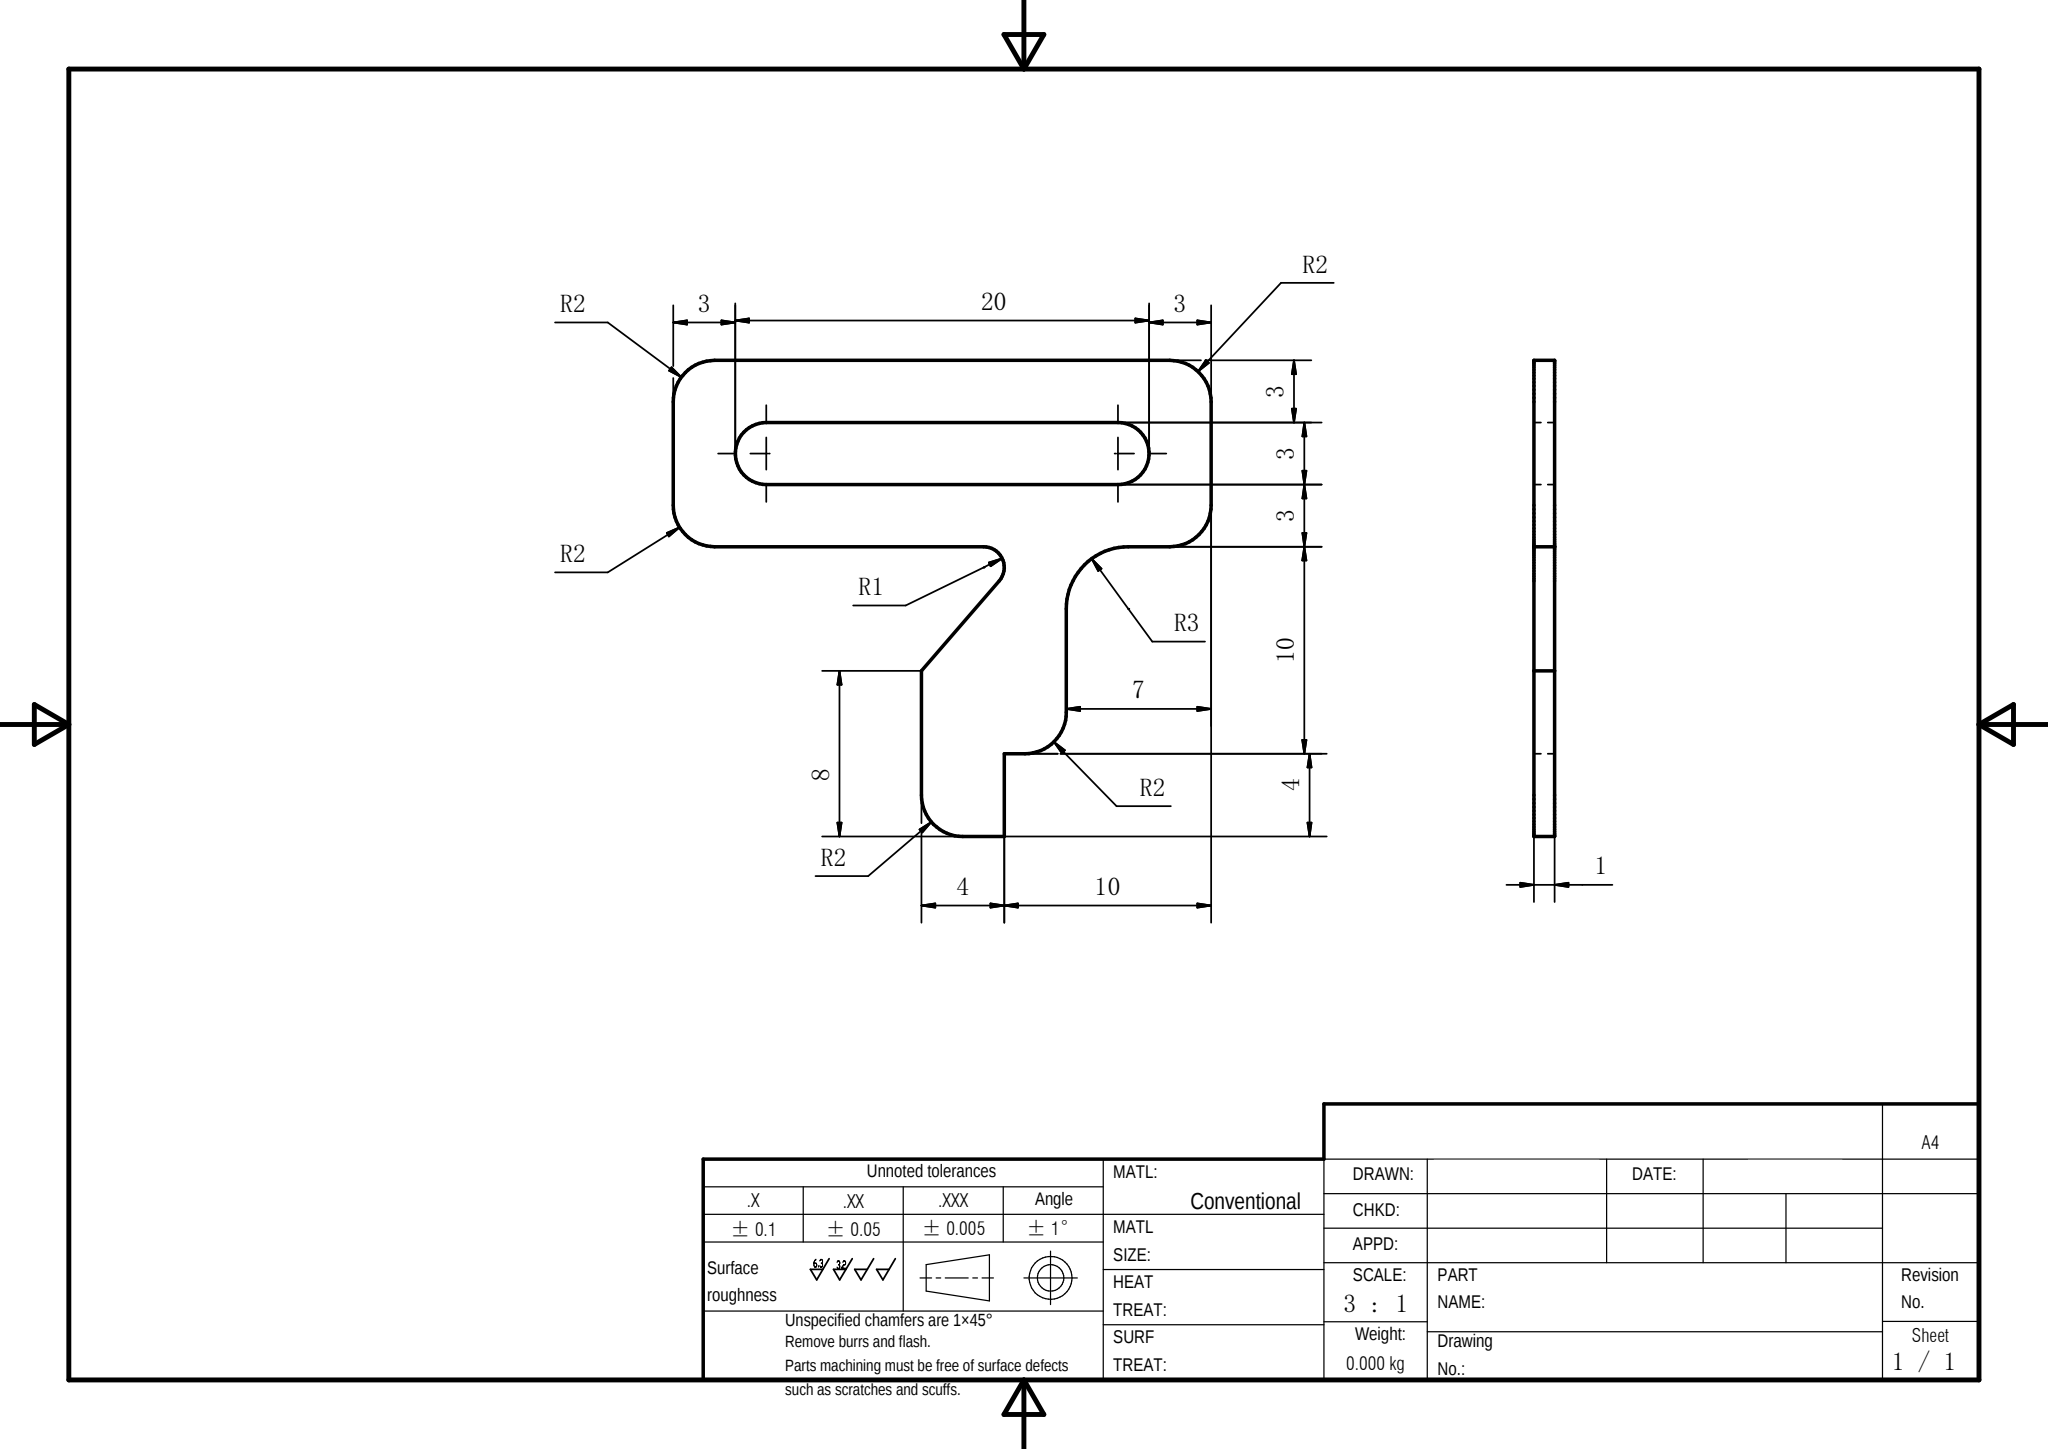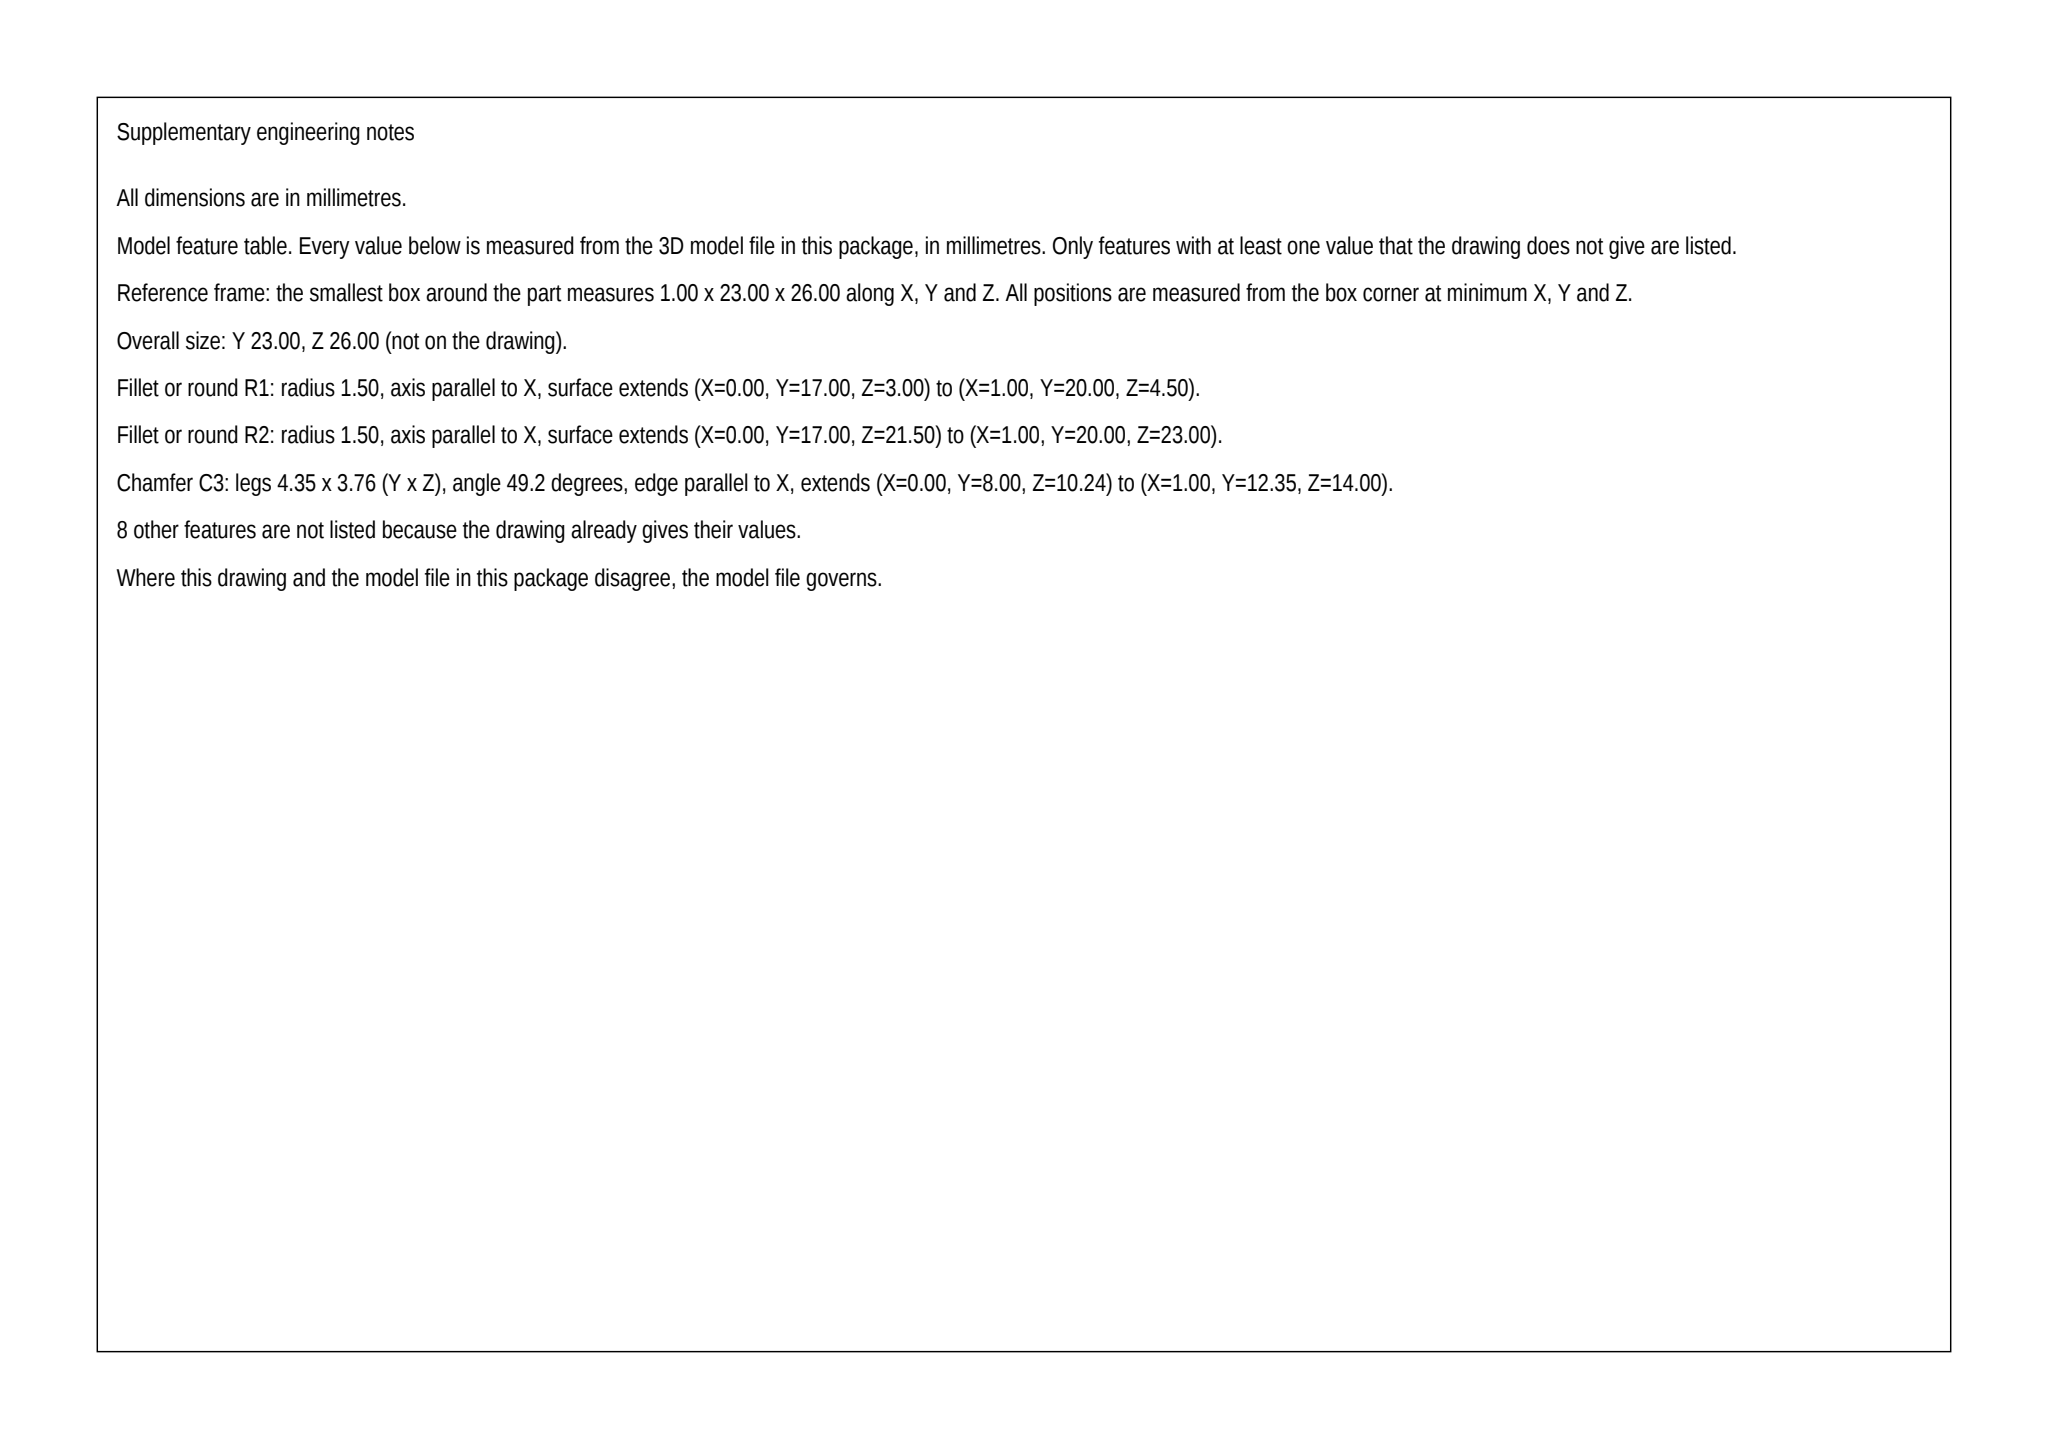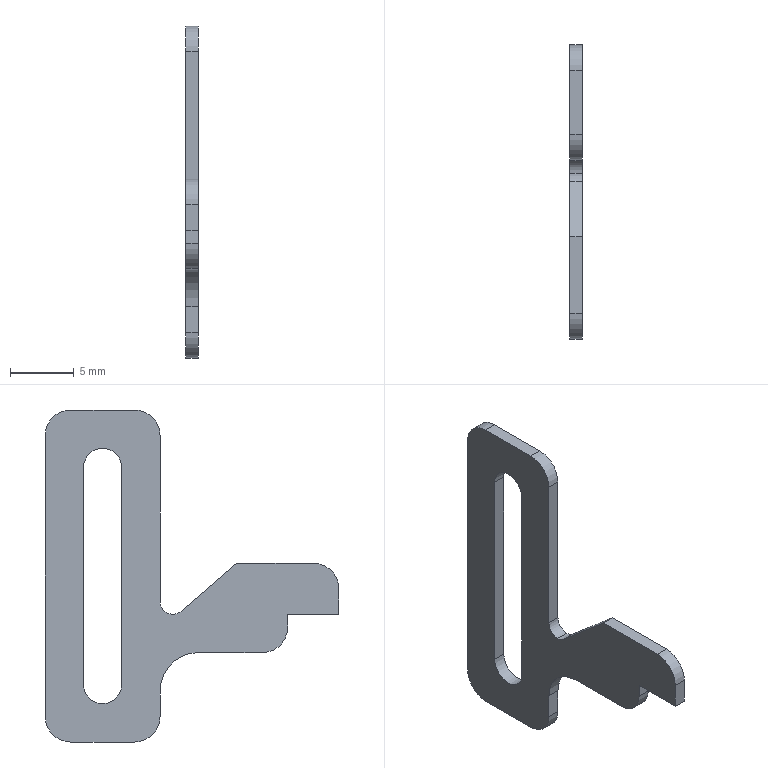Part | SolidWorks | mm | 1 solid | 27 faces | box 1 x 23 x 26 mm | volume 244 mm3 | plane 15 | cylinder 12 | commonest cylinder face diameters 4 x6 3 x3 2 x2 6 x1
STEP:
#1=CARTESIAN_POINT('',(1.,4.5,23.));
#2=VERTEX_POINT('',#1);
#3=CARTESIAN_POINT('',(1.,6.,21.5));
#4=VERTEX_POINT('',#3);
#5=CARTESIAN_POINT('',(1.,4.5,21.5));
#6=DIRECTION('',(-1.,0.,0.));
#7=DIRECTION('',(0.,0.,1.));
#8=AXIS2_PLACEMENT_3D('',#5,#6,#7);
#9=CIRCLE('',#8,1.5);
#10=EDGE_CURVE('',#2,#4,#9,.T.);
#11=ORIENTED_EDGE('',*,*,#10,.F.);
#12=CARTESIAN_POINT('',(0.,4.5,23.));
#13=VERTEX_POINT('',#12);
#14=CARTESIAN_POINT('',(1.,4.5,23.));
#15=DIRECTION('',(-1.,0.,0.));
#16=VECTOR('',#15,1000.);
#17=LINE('',#14,#16);
#18=EDGE_CURVE('',#2,#13,#17,.T.);
#19=ORIENTED_EDGE('',*,*,#18,.T.);
#20=CARTESIAN_POINT('',(0.,6.,21.5));
#21=VERTEX_POINT('',#20);
#22=CARTESIAN_POINT('',(0.,4.5,21.5));
#23=DIRECTION('',(-1.,0.,0.));
#24=DIRECTION('',(0.,0.,1.));
#25=AXIS2_PLACEMENT_3D('',#22,#23,#24);
#26=CIRCLE('',#25,1.5);
#27=EDGE_CURVE('',#13,#21,#26,.T.);
#28=ORIENTED_EDGE('',*,*,#27,.T.);
#29=CARTESIAN_POINT('',(1.,6.,21.5));
#30=DIRECTION('',(1.,0.,0.));
#31=VECTOR('',#30,1000.);
#32=LINE('',#29,#31);
#33=EDGE_CURVE('',#21,#4,#32,.T.);
#34=ORIENTED_EDGE('',*,*,#33,.T.);
#35=EDGE_LOOP('',(#11,#19,#28,#34));
#36=FACE_OUTER_BOUND('',#35,.T.);
#37=CARTESIAN_POINT('',(1.,4.5,21.5));
#38=DIRECTION('',(-1.,0.,0.));
#39=DIRECTION('',(0.,0.,1.));
#40=AXIS2_PLACEMENT_3D('',#37,#38,#39);
#41=CYLINDRICAL_SURFACE('',#40,1.5);
#42=ADVANCED_FACE('',(#36),#41,.F.);
#43=CARTESIAN_POINT('',(0.,-0.,11.));
#44=VERTEX_POINT('',#43);
#45=CARTESIAN_POINT('',(0.,-1.,10.));
#46=VERTEX_POINT('',#45);
#47=CARTESIAN_POINT('',(0.,-1.,11.));
#48=DIRECTION('',(-1.,0.,0.));
#49=DIRECTION('',(0.,0.,-1.));
#50=AXIS2_PLACEMENT_3D('',#47,#48,#49);
#51=CIRCLE('',#50,1.);
#52=EDGE_CURVE('',#44,#46,#51,.T.);
#53=ORIENTED_EDGE('',*,*,#52,.T.);
#54=CARTESIAN_POINT('',(1.,-1.,10.));
#55=VERTEX_POINT('',#54);
#56=CARTESIAN_POINT('',(0.,-1.,10.));
#57=DIRECTION('',(1.,0.,0.));
#58=VECTOR('',#57,1000.);
#59=LINE('',#56,#58);
#60=EDGE_CURVE('',#46,#55,#59,.T.);
#61=ORIENTED_EDGE('',*,*,#60,.T.);
#62=CARTESIAN_POINT('',(1.,-0.,11.));
#63=VERTEX_POINT('',#62);
#64=CARTESIAN_POINT('',(1.,-1.,11.));
#65=DIRECTION('',(-1.,0.,0.));
#66=DIRECTION('',(0.,0.,-1.));
#67=AXIS2_PLACEMENT_3D('',#64,#65,#66);
#68=CIRCLE('',#67,1.);
#69=EDGE_CURVE('',#63,#55,#68,.T.);
#70=ORIENTED_EDGE('',*,*,#69,.F.);
#71=CARTESIAN_POINT('',(0.,0.,11.));
#72=DIRECTION('',(1.,0.,0.));
#73=VECTOR('',#72,1000.);
#74=LINE('',#71,#73);
#75=EDGE_CURVE('',#44,#63,#74,.T.);
#76=ORIENTED_EDGE('',*,*,#75,.F.);
#77=EDGE_LOOP('',(#53,#61,#70,#76));
#78=FACE_OUTER_BOUND('',#77,.T.);
#79=CARTESIAN_POINT('',(0.,-1.,11.));
#80=DIRECTION('',(1.,0.,0.));
#81=DIRECTION('',(0.,0.,-1.));
#82=AXIS2_PLACEMENT_3D('',#79,#80,#81);
#83=CYLINDRICAL_SURFACE('',#82,1.);
#84=ADVANCED_FACE('',(#78),#83,.F.);
#85=CARTESIAN_POINT('',(0.,6.,4.5));
#86=VERTEX_POINT('',#85);
#87=CARTESIAN_POINT('',(0.,3.,4.5));
#88=VERTEX_POINT('',#87);
#89=CARTESIAN_POINT('',(0.,4.5,4.5));
#90=DIRECTION('',(-1.,0.,0.));
#91=DIRECTION('',(0.,0.,1.));
#92=AXIS2_PLACEMENT_3D('',#89,#90,#91);
#93=CIRCLE('',#92,1.5);
#94=EDGE_CURVE('',#86,#88,#93,.T.);
#95=ORIENTED_EDGE('',*,*,#94,.F.);
#96=CARTESIAN_POINT('',(0.,6.,13.));
#97=DIRECTION('',(0.,0.,-1.));
#98=VECTOR('',#97,1000.);
#99=LINE('',#96,#98);
#100=EDGE_CURVE('',#21,#86,#99,.T.);
#101=ORIENTED_EDGE('',*,*,#100,.F.);
#102=ORIENTED_EDGE('',*,*,#27,.F.);
#103=CARTESIAN_POINT('',(0.,3.,21.5));
#104=VERTEX_POINT('',#103);
#105=CARTESIAN_POINT('',(0.,4.5,21.5));
#106=DIRECTION('',(-1.,0.,0.));
#107=DIRECTION('',(0.,0.,1.));
#108=AXIS2_PLACEMENT_3D('',#105,#106,#107);
#109=CIRCLE('',#108,1.5);
#110=EDGE_CURVE('',#104,#13,#109,.T.);
#111=ORIENTED_EDGE('',*,*,#110,.F.);
#112=CARTESIAN_POINT('',(0.,3.,13.));
#113=DIRECTION('',(0.,0.,1.));
#114=VECTOR('',#113,1000.);
#115=LINE('',#112,#114);
#116=EDGE_CURVE('',#88,#104,#115,.T.);
#117=ORIENTED_EDGE('',*,*,#116,.F.);
#118=EDGE_LOOP('',(#95,#101,#102,#111,#117));
#119=FACE_BOUND('',#118,.T.);
#120=CARTESIAN_POINT('',(0.,7.,26.));
#121=VERTEX_POINT('',#120);
#122=CARTESIAN_POINT('',(0.,2.,26.));
#123=VERTEX_POINT('',#122);
#124=CARTESIAN_POINT('',(0.,4.5,26.));
#125=DIRECTION('',(0.,-1.,0.));
#126=VECTOR('',#125,1000.);
#127=LINE('',#124,#126);
#128=EDGE_CURVE('',#121,#123,#127,.T.);
#129=ORIENTED_EDGE('',*,*,#128,.F.);
#130=CARTESIAN_POINT('',(0.,9.,24.));
#131=VERTEX_POINT('',#130);
#132=CARTESIAN_POINT('',(0.,7.,24.));
#133=DIRECTION('',(1.,0.,0.));
#134=DIRECTION('',(0.,0.,-1.));
#135=AXIS2_PLACEMENT_3D('',#132,#133,#134);
#136=CIRCLE('',#135,2.);
#137=EDGE_CURVE('',#131,#121,#136,.T.);
#138=ORIENTED_EDGE('',*,*,#137,.F.);
#139=CARTESIAN_POINT('',(0.,9.,2.));
#140=VERTEX_POINT('',#139);
#141=CARTESIAN_POINT('',(0.,9.,13.));
#142=DIRECTION('',(0.,0.,1.));
#143=VECTOR('',#142,1000.);
#144=LINE('',#141,#143);
#145=EDGE_CURVE('',#140,#131,#144,.T.);
#146=ORIENTED_EDGE('',*,*,#145,.F.);
#147=CARTESIAN_POINT('',(0.,7.,0.));
#148=VERTEX_POINT('',#147);
#149=CARTESIAN_POINT('',(0.,7.,2.));
#150=DIRECTION('',(1.,0.,0.));
#151=DIRECTION('',(0.,0.,-1.));
#152=AXIS2_PLACEMENT_3D('',#149,#150,#151);
#153=CIRCLE('',#152,2.);
#154=EDGE_CURVE('',#148,#140,#153,.T.);
#155=ORIENTED_EDGE('',*,*,#154,.F.);
#156=CARTESIAN_POINT('',(0.,2.,0.));
#157=VERTEX_POINT('',#156);
#158=CARTESIAN_POINT('',(0.,4.5,0.));
#159=DIRECTION('',(0.,1.,0.));
#160=VECTOR('',#159,1000.);
#161=LINE('',#158,#160);
#162=EDGE_CURVE('',#157,#148,#161,.T.);
#163=ORIENTED_EDGE('',*,*,#162,.F.);
#164=CARTESIAN_POINT('',(0.,-0.,2.));
#165=VERTEX_POINT('',#164);
#166=CARTESIAN_POINT('',(0.,2.,2.));
#167=DIRECTION('',(1.,0.,0.));
#168=DIRECTION('',(0.,0.,-1.));
#169=AXIS2_PLACEMENT_3D('',#166,#167,#168);
#170=CIRCLE('',#169,2.);
#171=EDGE_CURVE('',#165,#157,#170,.T.);
#172=ORIENTED_EDGE('',*,*,#171,.F.);
#173=CARTESIAN_POINT('',(0.,-0.,4.));
#174=VERTEX_POINT('',#173);
#175=CARTESIAN_POINT('',(0.,-0.,13.));
#176=DIRECTION('',(0.,0.,-1.));
#177=VECTOR('',#176,1000.);
#178=LINE('',#175,#177);
#179=EDGE_CURVE('',#174,#165,#178,.T.);
#180=ORIENTED_EDGE('',*,*,#179,.F.);
#181=CARTESIAN_POINT('',(0.,-3.,7.));
#182=VERTEX_POINT('',#181);
#183=CARTESIAN_POINT('',(0.,-3.,4.));
#184=DIRECTION('',(-1.,0.,0.));
#185=DIRECTION('',(0.,0.,-1.));
#186=AXIS2_PLACEMENT_3D('',#183,#184,#185);
#187=CIRCLE('',#186,3.);
#188=EDGE_CURVE('',#182,#174,#187,.T.);
#189=ORIENTED_EDGE('',*,*,#188,.F.);
#190=CARTESIAN_POINT('',(0.,-8.,7.));
#191=VERTEX_POINT('',#190);
#192=CARTESIAN_POINT('',(0.,4.5,7.));
#193=DIRECTION('',(0.,1.,0.));
#194=VECTOR('',#193,1000.);
#195=LINE('',#192,#194);
#196=EDGE_CURVE('',#191,#182,#195,.T.);
#197=ORIENTED_EDGE('',*,*,#196,.F.);
#198=CARTESIAN_POINT('',(0.,-10.,9.));
#199=VERTEX_POINT('',#198);
#200=CARTESIAN_POINT('',(0.,-8.,9.));
#201=DIRECTION('',(1.,0.,0.));
#202=DIRECTION('',(0.,0.,-1.));
#203=AXIS2_PLACEMENT_3D('',#200,#201,#202);
#204=CIRCLE('',#203,2.);
#205=EDGE_CURVE('',#199,#191,#204,.T.);
#206=ORIENTED_EDGE('',*,*,#205,.F.);
#207=CARTESIAN_POINT('',(0.,-10.,10.));
#208=VERTEX_POINT('',#207);
#209=CARTESIAN_POINT('',(0.,-10.,13.));
#210=DIRECTION('',(0.,0.,-1.));
#211=VECTOR('',#210,1000.);
#212=LINE('',#209,#211);
#213=EDGE_CURVE('',#208,#199,#212,.T.);
#214=ORIENTED_EDGE('',*,*,#213,.F.);
#215=CARTESIAN_POINT('',(0.,-14.,10.));
#216=VERTEX_POINT('',#215);
#217=CARTESIAN_POINT('',(0.,4.5,10.));
#218=DIRECTION('',(0.,1.,0.));
#219=VECTOR('',#218,1000.);
#220=LINE('',#217,#219);
#221=EDGE_CURVE('',#216,#208,#220,.T.);
#222=ORIENTED_EDGE('',*,*,#221,.F.);
#223=CARTESIAN_POINT('',(0.,-14.,12.));
#224=VERTEX_POINT('',#223);
#225=CARTESIAN_POINT('',(0.,-14.,13.));
#226=DIRECTION('',(0.,0.,-1.));
#227=VECTOR('',#226,1000.);
#228=LINE('',#225,#227);
#229=EDGE_CURVE('',#224,#216,#228,.T.);
#230=ORIENTED_EDGE('',*,*,#229,.F.);
#231=CARTESIAN_POINT('',(0.,-12.,14.));
#232=VERTEX_POINT('',#231);
#233=CARTESIAN_POINT('',(0.,-12.,12.));
#234=DIRECTION('',(1.,0.,0.));
#235=DIRECTION('',(0.,0.,-1.));
#236=AXIS2_PLACEMENT_3D('',#233,#234,#235);
#237=CIRCLE('',#236,2.);
#238=EDGE_CURVE('',#232,#224,#237,.T.);
#239=ORIENTED_EDGE('',*,*,#238,.F.);
#240=CARTESIAN_POINT('',(0.,-6.,14.));
#241=VERTEX_POINT('',#240);
#242=CARTESIAN_POINT('',(0.,4.5,14.));
#243=DIRECTION('',(0.,-1.,0.));
#244=VECTOR('',#243,1000.);
#245=LINE('',#242,#244);
#246=EDGE_CURVE('',#241,#232,#245,.T.);
#247=ORIENTED_EDGE('',*,*,#246,.F.);
#248=CARTESIAN_POINT('',(0.,-1.654,10.243));
#249=VERTEX_POINT('',#248);
#250=CARTESIAN_POINT('',(0.,-1.654,10.243));
#251=DIRECTION('',(0.,-0.7566,0.6539));
#252=VECTOR('',#251,1000.);
#253=LINE('',#250,#252);
#254=EDGE_CURVE('',#249,#241,#253,.T.);
#255=ORIENTED_EDGE('',*,*,#254,.F.);
#256=CARTESIAN_POINT('',(0.,-1.,11.));
#257=DIRECTION('',(-1.,0.,0.));
#258=DIRECTION('',(0.,0.,-1.));
#259=AXIS2_PLACEMENT_3D('',#256,#257,#258);
#260=CIRCLE('',#259,1.);
#261=EDGE_CURVE('',#46,#249,#260,.T.);
#262=ORIENTED_EDGE('',*,*,#261,.F.);
#263=ORIENTED_EDGE('',*,*,#52,.F.);
#264=CARTESIAN_POINT('',(0.,-0.,24.));
#265=VERTEX_POINT('',#264);
#266=CARTESIAN_POINT('',(0.,-0.,13.));
#267=DIRECTION('',(0.,0.,-1.));
#268=VECTOR('',#267,1000.);
#269=LINE('',#266,#268);
#270=EDGE_CURVE('',#265,#44,#269,.T.);
#271=ORIENTED_EDGE('',*,*,#270,.F.);
#272=CARTESIAN_POINT('',(0.,2.,24.));
#273=DIRECTION('',(1.,0.,0.));
#274=DIRECTION('',(0.,0.,-1.));
#275=AXIS2_PLACEMENT_3D('',#272,#273,#274);
#276=CIRCLE('',#275,2.);
#277=EDGE_CURVE('',#123,#265,#276,.T.);
#278=ORIENTED_EDGE('',*,*,#277,.F.);
#279=EDGE_LOOP('',(#129,#138,#146,#155,#163,#172,#180,#189,#197,#206,#214,#222,#230,#239,#247,#255,#262,#263,#271,#278));
#280=FACE_OUTER_BOUND('',#279,.T.);
#281=CARTESIAN_POINT('',(0.,4.5,13.));
#282=DIRECTION('',(1.,0.,0.));
#283=DIRECTION('',(0.,0.,-1.));
#284=AXIS2_PLACEMENT_3D('',#281,#282,#283);
#285=PLANE('',#284);
#286=ADVANCED_FACE('',(#119,#280),#285,.F.);
#287=CARTESIAN_POINT('',(1.,3.,4.5));
#288=VERTEX_POINT('',#287);
#289=CARTESIAN_POINT('',(1.,3.,4.5));
#290=DIRECTION('',(1.,0.,0.));
#291=VECTOR('',#290,1000.);
#292=LINE('',#289,#291);
#293=EDGE_CURVE('',#88,#288,#292,.T.);
#294=ORIENTED_EDGE('',*,*,#293,.F.);
#295=ORIENTED_EDGE('',*,*,#116,.T.);
#296=CARTESIAN_POINT('',(1.,3.,21.5));
#297=VERTEX_POINT('',#296);
#298=CARTESIAN_POINT('',(1.,3.,21.5));
#299=DIRECTION('',(-1.,0.,0.));
#300=VECTOR('',#299,1000.);
#301=LINE('',#298,#300);
#302=EDGE_CURVE('',#297,#104,#301,.T.);
#303=ORIENTED_EDGE('',*,*,#302,.F.);
#304=CARTESIAN_POINT('',(1.,3.,4.5));
#305=DIRECTION('',(0.,-0.,1.));
#306=VECTOR('',#305,1000.);
#307=LINE('',#304,#306);
#308=EDGE_CURVE('',#288,#297,#307,.T.);
#309=ORIENTED_EDGE('',*,*,#308,.F.);
#310=EDGE_LOOP('',(#294,#295,#303,#309));
#311=FACE_OUTER_BOUND('',#310,.T.);
#312=CARTESIAN_POINT('',(1.,3.,4.5));
#313=DIRECTION('',(0.,-1.,-0.));
#314=DIRECTION('',(0.,0.,-1.));
#315=AXIS2_PLACEMENT_3D('',#312,#313,#314);
#316=PLANE('',#315);
#317=ADVANCED_FACE('',(#311),#316,.F.);
#318=CARTESIAN_POINT('',(1.,6.,4.5));
#319=VERTEX_POINT('',#318);
#320=CARTESIAN_POINT('',(1.,6.,4.5));
#321=DIRECTION('',(1.,0.,0.));
#322=VECTOR('',#321,1000.);
#323=LINE('',#320,#322);
#324=EDGE_CURVE('',#86,#319,#323,.T.);
#325=ORIENTED_EDGE('',*,*,#324,.F.);
#326=ORIENTED_EDGE('',*,*,#94,.T.);
#327=ORIENTED_EDGE('',*,*,#293,.T.);
#328=CARTESIAN_POINT('',(1.,4.5,4.5));
#329=DIRECTION('',(-1.,0.,0.));
#330=DIRECTION('',(0.,0.,1.));
#331=AXIS2_PLACEMENT_3D('',#328,#329,#330);
#332=CIRCLE('',#331,1.5);
#333=EDGE_CURVE('',#319,#288,#332,.T.);
#334=ORIENTED_EDGE('',*,*,#333,.F.);
#335=EDGE_LOOP('',(#325,#326,#327,#334));
#336=FACE_OUTER_BOUND('',#335,.T.);
#337=CARTESIAN_POINT('',(1.,4.5,4.5));
#338=DIRECTION('',(-1.,0.,0.));
#339=DIRECTION('',(0.,0.,1.));
#340=AXIS2_PLACEMENT_3D('',#337,#338,#339);
#341=CYLINDRICAL_SURFACE('',#340,1.5);
#342=ADVANCED_FACE('',(#336),#341,.F.);
#343=ORIENTED_EDGE('',*,*,#33,.F.);
#344=ORIENTED_EDGE('',*,*,#100,.T.);
#345=ORIENTED_EDGE('',*,*,#324,.T.);
#346=CARTESIAN_POINT('',(1.,6.,21.5));
#347=DIRECTION('',(0.,0.,-1.));
#348=VECTOR('',#347,1000.);
#349=LINE('',#346,#348);
#350=EDGE_CURVE('',#4,#319,#349,.T.);
#351=ORIENTED_EDGE('',*,*,#350,.F.);
#352=EDGE_LOOP('',(#343,#344,#345,#351));
#353=FACE_OUTER_BOUND('',#352,.T.);
#354=CARTESIAN_POINT('',(1.,6.,21.5));
#355=DIRECTION('',(0.,1.,0.));
#356=DIRECTION('',(0.,-0.,1.));
#357=AXIS2_PLACEMENT_3D('',#354,#355,#356);
#358=PLANE('',#357);
#359=ADVANCED_FACE('',(#353),#358,.F.);
#360=ORIENTED_EDGE('',*,*,#18,.F.);
#361=CARTESIAN_POINT('',(1.,4.5,21.5));
#362=DIRECTION('',(-1.,0.,0.));
#363=DIRECTION('',(0.,0.,1.));
#364=AXIS2_PLACEMENT_3D('',#361,#362,#363);
#365=CIRCLE('',#364,1.5);
#366=EDGE_CURVE('',#297,#2,#365,.T.);
#367=ORIENTED_EDGE('',*,*,#366,.F.);
#368=ORIENTED_EDGE('',*,*,#302,.T.);
#369=ORIENTED_EDGE('',*,*,#110,.T.);
#370=EDGE_LOOP('',(#360,#367,#368,#369));
#371=FACE_OUTER_BOUND('',#370,.T.);
#372=CARTESIAN_POINT('',(1.,4.5,21.5));
#373=DIRECTION('',(-1.,0.,0.));
#374=DIRECTION('',(0.,0.,1.));
#375=AXIS2_PLACEMENT_3D('',#372,#373,#374);
#376=CYLINDRICAL_SURFACE('',#375,1.5);
#377=ADVANCED_FACE('',(#371),#376,.F.);
#378=ORIENTED_EDGE('',*,*,#277,.T.);
#379=CARTESIAN_POINT('',(1.,-0.,24.));
#380=VERTEX_POINT('',#379);
#381=CARTESIAN_POINT('',(0.,-0.,24.));
#382=DIRECTION('',(1.,0.,0.));
#383=VECTOR('',#382,1000.);
#384=LINE('',#381,#383);
#385=EDGE_CURVE('',#265,#380,#384,.T.);
#386=ORIENTED_EDGE('',*,*,#385,.T.);
#387=CARTESIAN_POINT('',(1.,2.,26.));
#388=VERTEX_POINT('',#387);
#389=CARTESIAN_POINT('',(1.,2.,24.));
#390=DIRECTION('',(-1.,0.,0.));
#391=DIRECTION('',(0.,0.,-1.));
#392=AXIS2_PLACEMENT_3D('',#389,#390,#391);
#393=CIRCLE('',#392,2.);
#394=EDGE_CURVE('',#380,#388,#393,.T.);
#395=ORIENTED_EDGE('',*,*,#394,.T.);
#396=CARTESIAN_POINT('',(0.,2.,26.));
#397=DIRECTION('',(-1.,0.,0.));
#398=VECTOR('',#397,1000.);
#399=LINE('',#396,#398);
#400=EDGE_CURVE('',#388,#123,#399,.T.);
#401=ORIENTED_EDGE('',*,*,#400,.T.);
#402=EDGE_LOOP('',(#378,#386,#395,#401));
#403=FACE_OUTER_BOUND('',#402,.T.);
#404=CARTESIAN_POINT('',(0.,2.,24.));
#405=DIRECTION('',(1.,0.,0.));
#406=DIRECTION('',(0.,0.,-1.));
#407=AXIS2_PLACEMENT_3D('',#404,#405,#406);
#408=CYLINDRICAL_SURFACE('',#407,2.);
#409=ADVANCED_FACE('',(#403),#408,.T.);
#410=CARTESIAN_POINT('',(1.,7.,26.));
#411=VERTEX_POINT('',#410);
#412=CARTESIAN_POINT('',(0.,7.,26.));
#413=DIRECTION('',(-1.,0.,0.));
#414=VECTOR('',#413,1000.);
#415=LINE('',#412,#414);
#416=EDGE_CURVE('',#411,#121,#415,.T.);
#417=ORIENTED_EDGE('',*,*,#416,.T.);
#418=ORIENTED_EDGE('',*,*,#128,.T.);
#419=ORIENTED_EDGE('',*,*,#400,.F.);
#420=CARTESIAN_POINT('',(1.,9.,26.));
#421=DIRECTION('',(0.,1.,0.));
#422=VECTOR('',#421,1000.);
#423=LINE('',#420,#422);
#424=EDGE_CURVE('',#388,#411,#423,.T.);
#425=ORIENTED_EDGE('',*,*,#424,.T.);
#426=EDGE_LOOP('',(#417,#418,#419,#425));
#427=FACE_OUTER_BOUND('',#426,.T.);
#428=CARTESIAN_POINT('',(0.,9.,26.));
#429=DIRECTION('',(0.,-0.,1.));
#430=DIRECTION('',(0.,-1.,-0.));
#431=AXIS2_PLACEMENT_3D('',#428,#429,#430);
#432=PLANE('',#431);
#433=ADVANCED_FACE('',(#427),#432,.T.);
#434=ORIENTED_EDGE('',*,*,#137,.T.);
#435=ORIENTED_EDGE('',*,*,#416,.F.);
#436=CARTESIAN_POINT('',(1.,9.,24.));
#437=VERTEX_POINT('',#436);
#438=CARTESIAN_POINT('',(1.,7.,24.));
#439=DIRECTION('',(-1.,0.,0.));
#440=DIRECTION('',(0.,0.,-1.));
#441=AXIS2_PLACEMENT_3D('',#438,#439,#440);
#442=CIRCLE('',#441,2.);
#443=EDGE_CURVE('',#411,#437,#442,.T.);
#444=ORIENTED_EDGE('',*,*,#443,.T.);
#445=CARTESIAN_POINT('',(0.,9.,24.));
#446=DIRECTION('',(-1.,0.,0.));
#447=VECTOR('',#446,1000.);
#448=LINE('',#445,#447);
#449=EDGE_CURVE('',#437,#131,#448,.T.);
#450=ORIENTED_EDGE('',*,*,#449,.T.);
#451=EDGE_LOOP('',(#434,#435,#444,#450));
#452=FACE_OUTER_BOUND('',#451,.T.);
#453=CARTESIAN_POINT('',(0.,7.,24.));
#454=DIRECTION('',(1.,0.,0.));
#455=DIRECTION('',(0.,0.,-1.));
#456=AXIS2_PLACEMENT_3D('',#453,#454,#455);
#457=CYLINDRICAL_SURFACE('',#456,2.);
#458=ADVANCED_FACE('',(#452),#457,.T.);
#459=CARTESIAN_POINT('',(1.,9.,2.));
#460=VERTEX_POINT('',#459);
#461=CARTESIAN_POINT('',(0.,9.,2.));
#462=DIRECTION('',(-1.,0.,0.));
#463=VECTOR('',#462,1000.);
#464=LINE('',#461,#463);
#465=EDGE_CURVE('',#460,#140,#464,.T.);
#466=ORIENTED_EDGE('',*,*,#465,.T.);
#467=ORIENTED_EDGE('',*,*,#145,.T.);
#468=ORIENTED_EDGE('',*,*,#449,.F.);
#469=CARTESIAN_POINT('',(1.,9.,0.));
#470=DIRECTION('',(0.,0.,-1.));
#471=VECTOR('',#470,1000.);
#472=LINE('',#469,#471);
#473=EDGE_CURVE('',#437,#460,#472,.T.);
#474=ORIENTED_EDGE('',*,*,#473,.T.);
#475=EDGE_LOOP('',(#466,#467,#468,#474));
#476=FACE_OUTER_BOUND('',#475,.T.);
#477=CARTESIAN_POINT('',(0.,9.,0.));
#478=DIRECTION('',(0.,1.,0.));
#479=DIRECTION('',(0.,-0.,1.));
#480=AXIS2_PLACEMENT_3D('',#477,#478,#479);
#481=PLANE('',#480);
#482=ADVANCED_FACE('',(#476),#481,.T.);
#483=ORIENTED_EDGE('',*,*,#154,.T.);
#484=ORIENTED_EDGE('',*,*,#465,.F.);
#485=CARTESIAN_POINT('',(1.,7.,0.));
#486=VERTEX_POINT('',#485);
#487=CARTESIAN_POINT('',(1.,7.,2.));
#488=DIRECTION('',(-1.,0.,0.));
#489=DIRECTION('',(0.,0.,-1.));
#490=AXIS2_PLACEMENT_3D('',#487,#488,#489);
#491=CIRCLE('',#490,2.);
#492=EDGE_CURVE('',#460,#486,#491,.T.);
#493=ORIENTED_EDGE('',*,*,#492,.T.);
#494=CARTESIAN_POINT('',(0.,7.,0.));
#495=DIRECTION('',(-1.,0.,0.));
#496=VECTOR('',#495,1000.);
#497=LINE('',#494,#496);
#498=EDGE_CURVE('',#486,#148,#497,.T.);
#499=ORIENTED_EDGE('',*,*,#498,.T.);
#500=EDGE_LOOP('',(#483,#484,#493,#499));
#501=FACE_OUTER_BOUND('',#500,.T.);
#502=CARTESIAN_POINT('',(0.,7.,2.));
#503=DIRECTION('',(1.,0.,0.));
#504=DIRECTION('',(0.,0.,-1.));
#505=AXIS2_PLACEMENT_3D('',#502,#503,#504);
#506=CYLINDRICAL_SURFACE('',#505,2.);
#507=ADVANCED_FACE('',(#501),#506,.T.);
#508=CARTESIAN_POINT('',(1.,2.,0.));
#509=VERTEX_POINT('',#508);
#510=CARTESIAN_POINT('',(0.,2.,0.));
#511=DIRECTION('',(-1.,0.,0.));
#512=VECTOR('',#511,1000.);
#513=LINE('',#510,#512);
#514=EDGE_CURVE('',#509,#157,#513,.T.);
#515=ORIENTED_EDGE('',*,*,#514,.T.);
#516=ORIENTED_EDGE('',*,*,#162,.T.);
#517=ORIENTED_EDGE('',*,*,#498,.F.);
#518=CARTESIAN_POINT('',(1.,0.,0.));
#519=DIRECTION('',(0.,-1.,0.));
#520=VECTOR('',#519,1000.);
#521=LINE('',#518,#520);
#522=EDGE_CURVE('',#486,#509,#521,.T.);
#523=ORIENTED_EDGE('',*,*,#522,.T.);
#524=EDGE_LOOP('',(#515,#516,#517,#523));
#525=FACE_OUTER_BOUND('',#524,.T.);
#526=CARTESIAN_POINT('',(0.,0.,0.));
#527=DIRECTION('',(0.,0.,-1.));
#528=DIRECTION('',(-1.,0.,0.));
#529=AXIS2_PLACEMENT_3D('',#526,#527,#528);
#530=PLANE('',#529);
#531=ADVANCED_FACE('',(#525),#530,.T.);
#532=ORIENTED_EDGE('',*,*,#171,.T.);
#533=ORIENTED_EDGE('',*,*,#514,.F.);
#534=CARTESIAN_POINT('',(1.,-0.,2.));
#535=VERTEX_POINT('',#534);
#536=CARTESIAN_POINT('',(1.,2.,2.));
#537=DIRECTION('',(-1.,0.,0.));
#538=DIRECTION('',(0.,0.,-1.));
#539=AXIS2_PLACEMENT_3D('',#536,#537,#538);
#540=CIRCLE('',#539,2.);
#541=EDGE_CURVE('',#509,#535,#540,.T.);
#542=ORIENTED_EDGE('',*,*,#541,.T.);
#543=CARTESIAN_POINT('',(0.,0.,2.));
#544=DIRECTION('',(-1.,0.,0.));
#545=VECTOR('',#544,1000.);
#546=LINE('',#543,#545);
#547=EDGE_CURVE('',#535,#165,#546,.T.);
#548=ORIENTED_EDGE('',*,*,#547,.T.);
#549=EDGE_LOOP('',(#532,#533,#542,#548));
#550=FACE_OUTER_BOUND('',#549,.T.);
#551=CARTESIAN_POINT('',(0.,2.,2.));
#552=DIRECTION('',(1.,0.,0.));
#553=DIRECTION('',(0.,0.,-1.));
#554=AXIS2_PLACEMENT_3D('',#551,#552,#553);
#555=CYLINDRICAL_SURFACE('',#554,2.);
#556=ADVANCED_FACE('',(#550),#555,.T.);
#557=ORIENTED_EDGE('',*,*,#547,.F.);
#558=CARTESIAN_POINT('',(1.,-0.,4.));
#559=VERTEX_POINT('',#558);
#560=CARTESIAN_POINT('',(1.,-0.,7.));
#561=DIRECTION('',(0.,-0.,1.));
#562=VECTOR('',#561,1000.);
#563=LINE('',#560,#562);
#564=EDGE_CURVE('',#535,#559,#563,.T.);
#565=ORIENTED_EDGE('',*,*,#564,.T.);
#566=CARTESIAN_POINT('',(0.,-0.,4.));
#567=DIRECTION('',(-1.,0.,0.));
#568=VECTOR('',#567,1000.);
#569=LINE('',#566,#568);
#570=EDGE_CURVE('',#559,#174,#569,.T.);
#571=ORIENTED_EDGE('',*,*,#570,.T.);
#572=ORIENTED_EDGE('',*,*,#179,.T.);
#573=EDGE_LOOP('',(#557,#565,#571,#572));
#574=FACE_OUTER_BOUND('',#573,.T.);
#575=CARTESIAN_POINT('',(0.,-0.,7.));
#576=DIRECTION('',(0.,-1.,-0.));
#577=DIRECTION('',(0.,0.,-1.));
#578=AXIS2_PLACEMENT_3D('',#575,#576,#577);
#579=PLANE('',#578);
#580=ADVANCED_FACE('',(#574),#579,.T.);
#581=ORIENTED_EDGE('',*,*,#570,.F.);
#582=CARTESIAN_POINT('',(1.,-3.,7.));
#583=VERTEX_POINT('',#582);
#584=CARTESIAN_POINT('',(1.,-3.,4.));
#585=DIRECTION('',(-1.,0.,0.));
#586=DIRECTION('',(0.,0.,-1.));
#587=AXIS2_PLACEMENT_3D('',#584,#585,#586);
#588=CIRCLE('',#587,3.);
#589=EDGE_CURVE('',#583,#559,#588,.T.);
#590=ORIENTED_EDGE('',*,*,#589,.F.);
#591=CARTESIAN_POINT('',(0.,-3.,7.));
#592=DIRECTION('',(1.,0.,0.));
#593=VECTOR('',#592,1000.);
#594=LINE('',#591,#593);
#595=EDGE_CURVE('',#182,#583,#594,.T.);
#596=ORIENTED_EDGE('',*,*,#595,.F.);
#597=ORIENTED_EDGE('',*,*,#188,.T.);
#598=EDGE_LOOP('',(#581,#590,#596,#597));
#599=FACE_OUTER_BOUND('',#598,.T.);
#600=CARTESIAN_POINT('',(0.,-3.,4.));
#601=DIRECTION('',(1.,0.,0.));
#602=DIRECTION('',(0.,0.,-1.));
#603=AXIS2_PLACEMENT_3D('',#600,#601,#602);
#604=CYLINDRICAL_SURFACE('',#603,3.);
#605=ADVANCED_FACE('',(#599),#604,.F.);
#606=CARTESIAN_POINT('',(1.,-8.,7.));
#607=VERTEX_POINT('',#606);
#608=CARTESIAN_POINT('',(0.,-8.,7.));
#609=DIRECTION('',(-1.,0.,0.));
#610=VECTOR('',#609,1000.);
#611=LINE('',#608,#610);
#612=EDGE_CURVE('',#607,#191,#611,.T.);
#613=ORIENTED_EDGE('',*,*,#612,.T.);
#614=ORIENTED_EDGE('',*,*,#196,.T.);
#615=ORIENTED_EDGE('',*,*,#595,.T.);
#616=CARTESIAN_POINT('',(1.,-10.,7.));
#617=DIRECTION('',(0.,-1.,-0.));
#618=VECTOR('',#617,1000.);
#619=LINE('',#616,#618);
#620=EDGE_CURVE('',#583,#607,#619,.T.);
#621=ORIENTED_EDGE('',*,*,#620,.T.);
#622=EDGE_LOOP('',(#613,#614,#615,#621));
#623=FACE_OUTER_BOUND('',#622,.T.);
#624=CARTESIAN_POINT('',(0.,-10.,7.));
#625=DIRECTION('',(0.,0.,-1.));
#626=DIRECTION('',(0.,1.,0.));
#627=AXIS2_PLACEMENT_3D('',#624,#625,#626);
#628=PLANE('',#627);
#629=ADVANCED_FACE('',(#623),#628,.T.);
#630=ORIENTED_EDGE('',*,*,#205,.T.);
#631=ORIENTED_EDGE('',*,*,#612,.F.);
#632=CARTESIAN_POINT('',(1.,-10.,9.));
#633=VERTEX_POINT('',#632);
#634=CARTESIAN_POINT('',(1.,-8.,9.));
#635=DIRECTION('',(-1.,0.,0.));
#636=DIRECTION('',(0.,0.,-1.));
#637=AXIS2_PLACEMENT_3D('',#634,#635,#636);
#638=CIRCLE('',#637,2.);
#639=EDGE_CURVE('',#607,#633,#638,.T.);
#640=ORIENTED_EDGE('',*,*,#639,.T.);
#641=CARTESIAN_POINT('',(0.,-10.,9.));
#642=DIRECTION('',(-1.,0.,0.));
#643=VECTOR('',#642,1000.);
#644=LINE('',#641,#643);
#645=EDGE_CURVE('',#633,#199,#644,.T.);
#646=ORIENTED_EDGE('',*,*,#645,.T.);
#647=EDGE_LOOP('',(#630,#631,#640,#646));
#648=FACE_OUTER_BOUND('',#647,.T.);
#649=CARTESIAN_POINT('',(0.,-8.,9.));
#650=DIRECTION('',(1.,0.,0.));
#651=DIRECTION('',(0.,0.,-1.));
#652=AXIS2_PLACEMENT_3D('',#649,#650,#651);
#653=CYLINDRICAL_SURFACE('',#652,2.);
#654=ADVANCED_FACE('',(#648),#653,.T.);
#655=CARTESIAN_POINT('',(1.,-10.,10.));
#656=VERTEX_POINT('',#655);
#657=CARTESIAN_POINT('',(0.,-10.,10.));
#658=DIRECTION('',(-1.,0.,0.));
#659=VECTOR('',#658,1000.);
#660=LINE('',#657,#659);
#661=EDGE_CURVE('',#656,#208,#660,.T.);
#662=ORIENTED_EDGE('',*,*,#661,.T.);
#663=ORIENTED_EDGE('',*,*,#213,.T.);
#664=ORIENTED_EDGE('',*,*,#645,.F.);
#665=CARTESIAN_POINT('',(1.,-10.,10.));
#666=DIRECTION('',(0.,0.,1.));
#667=VECTOR('',#666,1000.);
#668=LINE('',#665,#667);
#669=EDGE_CURVE('',#633,#656,#668,.T.);
#670=ORIENTED_EDGE('',*,*,#669,.T.);
#671=EDGE_LOOP('',(#662,#663,#664,#670));
#672=FACE_OUTER_BOUND('',#671,.T.);
#673=CARTESIAN_POINT('',(0.,-10.,10.));
#674=DIRECTION('',(0.,-1.,0.));
#675=DIRECTION('',(0.,0.,-1.));
#676=AXIS2_PLACEMENT_3D('',#673,#674,#675);
#677=PLANE('',#676);
#678=ADVANCED_FACE('',(#672),#677,.T.);
#679=CARTESIAN_POINT('',(1.,-14.,10.));
#680=VERTEX_POINT('',#679);
#681=CARTESIAN_POINT('',(1.,-14.,10.));
#682=DIRECTION('',(0.,-1.,0.));
#683=VECTOR('',#682,1000.);
#684=LINE('',#681,#683);
#685=EDGE_CURVE('',#656,#680,#684,.T.);
#686=ORIENTED_EDGE('',*,*,#685,.T.);
#687=CARTESIAN_POINT('',(0.,-14.,10.));
#688=DIRECTION('',(-1.,0.,0.));
#689=VECTOR('',#688,1000.);
#690=LINE('',#687,#689);
#691=EDGE_CURVE('',#680,#216,#690,.T.);
#692=ORIENTED_EDGE('',*,*,#691,.T.);
#693=ORIENTED_EDGE('',*,*,#221,.T.);
#694=ORIENTED_EDGE('',*,*,#661,.F.);
#695=EDGE_LOOP('',(#686,#692,#693,#694));
#696=FACE_OUTER_BOUND('',#695,.T.);
#697=CARTESIAN_POINT('',(0.,-14.,10.));
#698=DIRECTION('',(0.,0.,-1.));
#699=DIRECTION('',(-1.,0.,0.));
#700=AXIS2_PLACEMENT_3D('',#697,#698,#699);
#701=PLANE('',#700);
#702=ADVANCED_FACE('',(#696),#701,.T.);
#703=ORIENTED_EDGE('',*,*,#691,.F.);
#704=CARTESIAN_POINT('',(1.,-14.,12.));
#705=VERTEX_POINT('',#704);
#706=CARTESIAN_POINT('',(1.,-14.,14.));
#707=DIRECTION('',(0.,-0.,1.));
#708=VECTOR('',#707,1000.);
#709=LINE('',#706,#708);
#710=EDGE_CURVE('',#680,#705,#709,.T.);
#711=ORIENTED_EDGE('',*,*,#710,.T.);
#712=CARTESIAN_POINT('',(0.,-14.,12.));
#713=DIRECTION('',(-1.,0.,0.));
#714=VECTOR('',#713,1000.);
#715=LINE('',#712,#714);
#716=EDGE_CURVE('',#705,#224,#715,.T.);
#717=ORIENTED_EDGE('',*,*,#716,.T.);
#718=ORIENTED_EDGE('',*,*,#229,.T.);
#719=EDGE_LOOP('',(#703,#711,#717,#718));
#720=FACE_OUTER_BOUND('',#719,.T.);
#721=CARTESIAN_POINT('',(0.,-14.,14.));
#722=DIRECTION('',(0.,-1.,-0.));
#723=DIRECTION('',(0.,0.,-1.));
#724=AXIS2_PLACEMENT_3D('',#721,#722,#723);
#725=PLANE('',#724);
#726=ADVANCED_FACE('',(#720),#725,.T.);
#727=ORIENTED_EDGE('',*,*,#238,.T.);
#728=ORIENTED_EDGE('',*,*,#716,.F.);
#729=CARTESIAN_POINT('',(1.,-12.,14.));
#730=VERTEX_POINT('',#729);
#731=CARTESIAN_POINT('',(1.,-12.,12.));
#732=DIRECTION('',(-1.,0.,0.));
#733=DIRECTION('',(0.,0.,-1.));
#734=AXIS2_PLACEMENT_3D('',#731,#732,#733);
#735=CIRCLE('',#734,2.);
#736=EDGE_CURVE('',#705,#730,#735,.T.);
#737=ORIENTED_EDGE('',*,*,#736,.T.);
#738=CARTESIAN_POINT('',(0.,-12.,14.));
#739=DIRECTION('',(-1.,0.,0.));
#740=VECTOR('',#739,1000.);
#741=LINE('',#738,#740);
#742=EDGE_CURVE('',#730,#232,#741,.T.);
#743=ORIENTED_EDGE('',*,*,#742,.T.);
#744=EDGE_LOOP('',(#727,#728,#737,#743));
#745=FACE_OUTER_BOUND('',#744,.T.);
#746=CARTESIAN_POINT('',(0.,-12.,12.));
#747=DIRECTION('',(1.,0.,0.));
#748=DIRECTION('',(0.,0.,-1.));
#749=AXIS2_PLACEMENT_3D('',#746,#747,#748);
#750=CYLINDRICAL_SURFACE('',#749,2.);
#751=ADVANCED_FACE('',(#745),#750,.T.);
#752=CARTESIAN_POINT('',(1.,-6.,14.));
#753=VERTEX_POINT('',#752);
#754=CARTESIAN_POINT('',(0.,-6.,14.));
#755=DIRECTION('',(-1.,0.,0.));
#756=VECTOR('',#755,1000.);
#757=LINE('',#754,#756);
#758=EDGE_CURVE('',#753,#241,#757,.T.);
#759=ORIENTED_EDGE('',*,*,#758,.T.);
#760=ORIENTED_EDGE('',*,*,#246,.T.);
#761=ORIENTED_EDGE('',*,*,#742,.F.);
#762=CARTESIAN_POINT('',(1.,-6.,14.));
#763=DIRECTION('',(0.,1.,0.));
#764=VECTOR('',#763,1000.);
#765=LINE('',#762,#764);
#766=EDGE_CURVE('',#730,#753,#765,.T.);
#767=ORIENTED_EDGE('',*,*,#766,.T.);
#768=EDGE_LOOP('',(#759,#760,#761,#767));
#769=FACE_OUTER_BOUND('',#768,.T.);
#770=CARTESIAN_POINT('',(0.,-6.,14.));
#771=DIRECTION('',(0.,-0.,1.));
#772=DIRECTION('',(0.,-1.,-0.));
#773=AXIS2_PLACEMENT_3D('',#770,#771,#772);
#774=PLANE('',#773);
#775=ADVANCED_FACE('',(#769),#774,.T.);
#776=CARTESIAN_POINT('',(1.,-1.654,10.243));
#777=VERTEX_POINT('',#776);
#778=CARTESIAN_POINT('',(1.,-1.654,10.243));
#779=DIRECTION('',(0.,0.7566,-0.6539));
#780=VECTOR('',#779,1000.);
#781=LINE('',#778,#780);
#782=EDGE_CURVE('',#753,#777,#781,.T.);
#783=ORIENTED_EDGE('',*,*,#782,.T.);
#784=CARTESIAN_POINT('',(0.,-1.654,10.243));
#785=DIRECTION('',(-1.,0.,0.));
#786=VECTOR('',#785,1000.);
#787=LINE('',#784,#786);
#788=EDGE_CURVE('',#777,#249,#787,.T.);
#789=ORIENTED_EDGE('',*,*,#788,.T.);
#790=ORIENTED_EDGE('',*,*,#254,.T.);
#791=ORIENTED_EDGE('',*,*,#758,.F.);
#792=EDGE_LOOP('',(#783,#789,#790,#791));
#793=FACE_OUTER_BOUND('',#792,.T.);
#794=CARTESIAN_POINT('',(0.,-1.654,10.243));
#795=DIRECTION('',(0.,0.6539,0.7566));
#796=DIRECTION('',(0.,-0.7566,0.6539));
#797=AXIS2_PLACEMENT_3D('',#794,#795,#796);
#798=PLANE('',#797);
#799=ADVANCED_FACE('',(#793),#798,.T.);
#800=ORIENTED_EDGE('',*,*,#60,.F.);
#801=ORIENTED_EDGE('',*,*,#261,.T.);
#802=ORIENTED_EDGE('',*,*,#788,.F.);
#803=CARTESIAN_POINT('',(1.,-1.,11.));
#804=DIRECTION('',(-1.,0.,0.));
#805=DIRECTION('',(0.,0.,-1.));
#806=AXIS2_PLACEMENT_3D('',#803,#804,#805);
#807=CIRCLE('',#806,1.);
#808=EDGE_CURVE('',#55,#777,#807,.T.);
#809=ORIENTED_EDGE('',*,*,#808,.F.);
#810=EDGE_LOOP('',(#800,#801,#802,#809));
#811=FACE_OUTER_BOUND('',#810,.T.);
#812=CARTESIAN_POINT('',(0.,-1.,11.));
#813=DIRECTION('',(1.,0.,0.));
#814=DIRECTION('',(0.,0.,-1.));
#815=AXIS2_PLACEMENT_3D('',#812,#813,#814);
#816=CYLINDRICAL_SURFACE('',#815,1.);
#817=ADVANCED_FACE('',(#811),#816,.F.);
#818=ORIENTED_EDGE('',*,*,#75,.T.);
#819=CARTESIAN_POINT('',(1.,-0.,26.));
#820=DIRECTION('',(0.,-0.,1.));
#821=VECTOR('',#820,1000.);
#822=LINE('',#819,#821);
#823=EDGE_CURVE('',#63,#380,#822,.T.);
#824=ORIENTED_EDGE('',*,*,#823,.T.);
#825=ORIENTED_EDGE('',*,*,#385,.F.);
#826=ORIENTED_EDGE('',*,*,#270,.T.);
#827=EDGE_LOOP('',(#818,#824,#825,#826));
#828=FACE_OUTER_BOUND('',#827,.T.);
#829=CARTESIAN_POINT('',(0.,-0.,26.));
#830=DIRECTION('',(0.,-1.,-0.));
#831=DIRECTION('',(0.,0.,-1.));
#832=AXIS2_PLACEMENT_3D('',#829,#830,#831);
#833=PLANE('',#832);
#834=ADVANCED_FACE('',(#828),#833,.T.);
#835=ORIENTED_EDGE('',*,*,#350,.T.);
#836=ORIENTED_EDGE('',*,*,#333,.T.);
#837=ORIENTED_EDGE('',*,*,#308,.T.);
#838=ORIENTED_EDGE('',*,*,#366,.T.);
#839=ORIENTED_EDGE('',*,*,#10,.T.);
#840=EDGE_LOOP('',(#835,#836,#837,#838,#839));
#841=FACE_BOUND('',#840,.T.);
#842=ORIENTED_EDGE('',*,*,#443,.F.);
#843=ORIENTED_EDGE('',*,*,#424,.F.);
#844=ORIENTED_EDGE('',*,*,#394,.F.);
#845=ORIENTED_EDGE('',*,*,#823,.F.);
#846=ORIENTED_EDGE('',*,*,#69,.T.);
#847=ORIENTED_EDGE('',*,*,#808,.T.);
#848=ORIENTED_EDGE('',*,*,#782,.F.);
#849=ORIENTED_EDGE('',*,*,#766,.F.);
#850=ORIENTED_EDGE('',*,*,#736,.F.);
#851=ORIENTED_EDGE('',*,*,#710,.F.);
#852=ORIENTED_EDGE('',*,*,#685,.F.);
#853=ORIENTED_EDGE('',*,*,#669,.F.);
#854=ORIENTED_EDGE('',*,*,#639,.F.);
#855=ORIENTED_EDGE('',*,*,#620,.F.);
#856=ORIENTED_EDGE('',*,*,#589,.T.);
#857=ORIENTED_EDGE('',*,*,#564,.F.);
#858=ORIENTED_EDGE('',*,*,#541,.F.);
#859=ORIENTED_EDGE('',*,*,#522,.F.);
#860=ORIENTED_EDGE('',*,*,#492,.F.);
#861=ORIENTED_EDGE('',*,*,#473,.F.);
#862=EDGE_LOOP('',(#842,#843,#844,#845,#846,#847,#848,#849,#850,#851,#852,#853,#854,#855,#856,#857,#858,#859,#860,#861));
#863=FACE_OUTER_BOUND('',#862,.T.);
#864=CARTESIAN_POINT('',(1.,4.5,13.));
#865=DIRECTION('',(1.,0.,0.));
#866=DIRECTION('',(0.,0.,-1.));
#867=AXIS2_PLACEMENT_3D('',#864,#865,#866);
#868=PLANE('',#867);
#869=ADVANCED_FACE('',(#841,#863),#868,.T.);
#870=CLOSED_SHELL('',(#42,#84,#286,#317,#342,#359,#377,#409,#433,#458,#482,#507,#531,#556,#580,#605,#629,#654,#678,#702,#726,#751,#775,#799,#817,#834,#869));
#871=MANIFOLD_SOLID_BREP('',#870);
#872=CARTESIAN_POINT('',(0.,0.,0.));
#873=DIRECTION('',(0.,0.,1.));
#874=DIRECTION('',(1.,0.,0.));
#875=AXIS2_PLACEMENT_3D('',#872,#873,#874);
#876=(LENGTH_UNIT()NAMED_UNIT(*)SI_UNIT(.MILLI.,.METRE.));
#877=UNCERTAINTY_MEASURE_WITH_UNIT(LENGTH_MEASURE(0.00001),#876,'','');
#878=(NAMED_UNIT(*)PLANE_ANGLE_UNIT()SI_UNIT($,.RADIAN.));
#879=(NAMED_UNIT(*)SI_UNIT($,.STERADIAN.)SOLID_ANGLE_UNIT());
#880=(GEOMETRIC_REPRESENTATION_CONTEXT(3)GLOBAL_UNCERTAINTY_ASSIGNED_CONTEXT((#877))GLOBAL_UNIT_ASSIGNED_CONTEXT((#876,#878,#879))REPRESENTATION_CONTEXT('',''));
#881=ADVANCED_BREP_SHAPE_REPRESENTATION('',(#871,#875),#880);